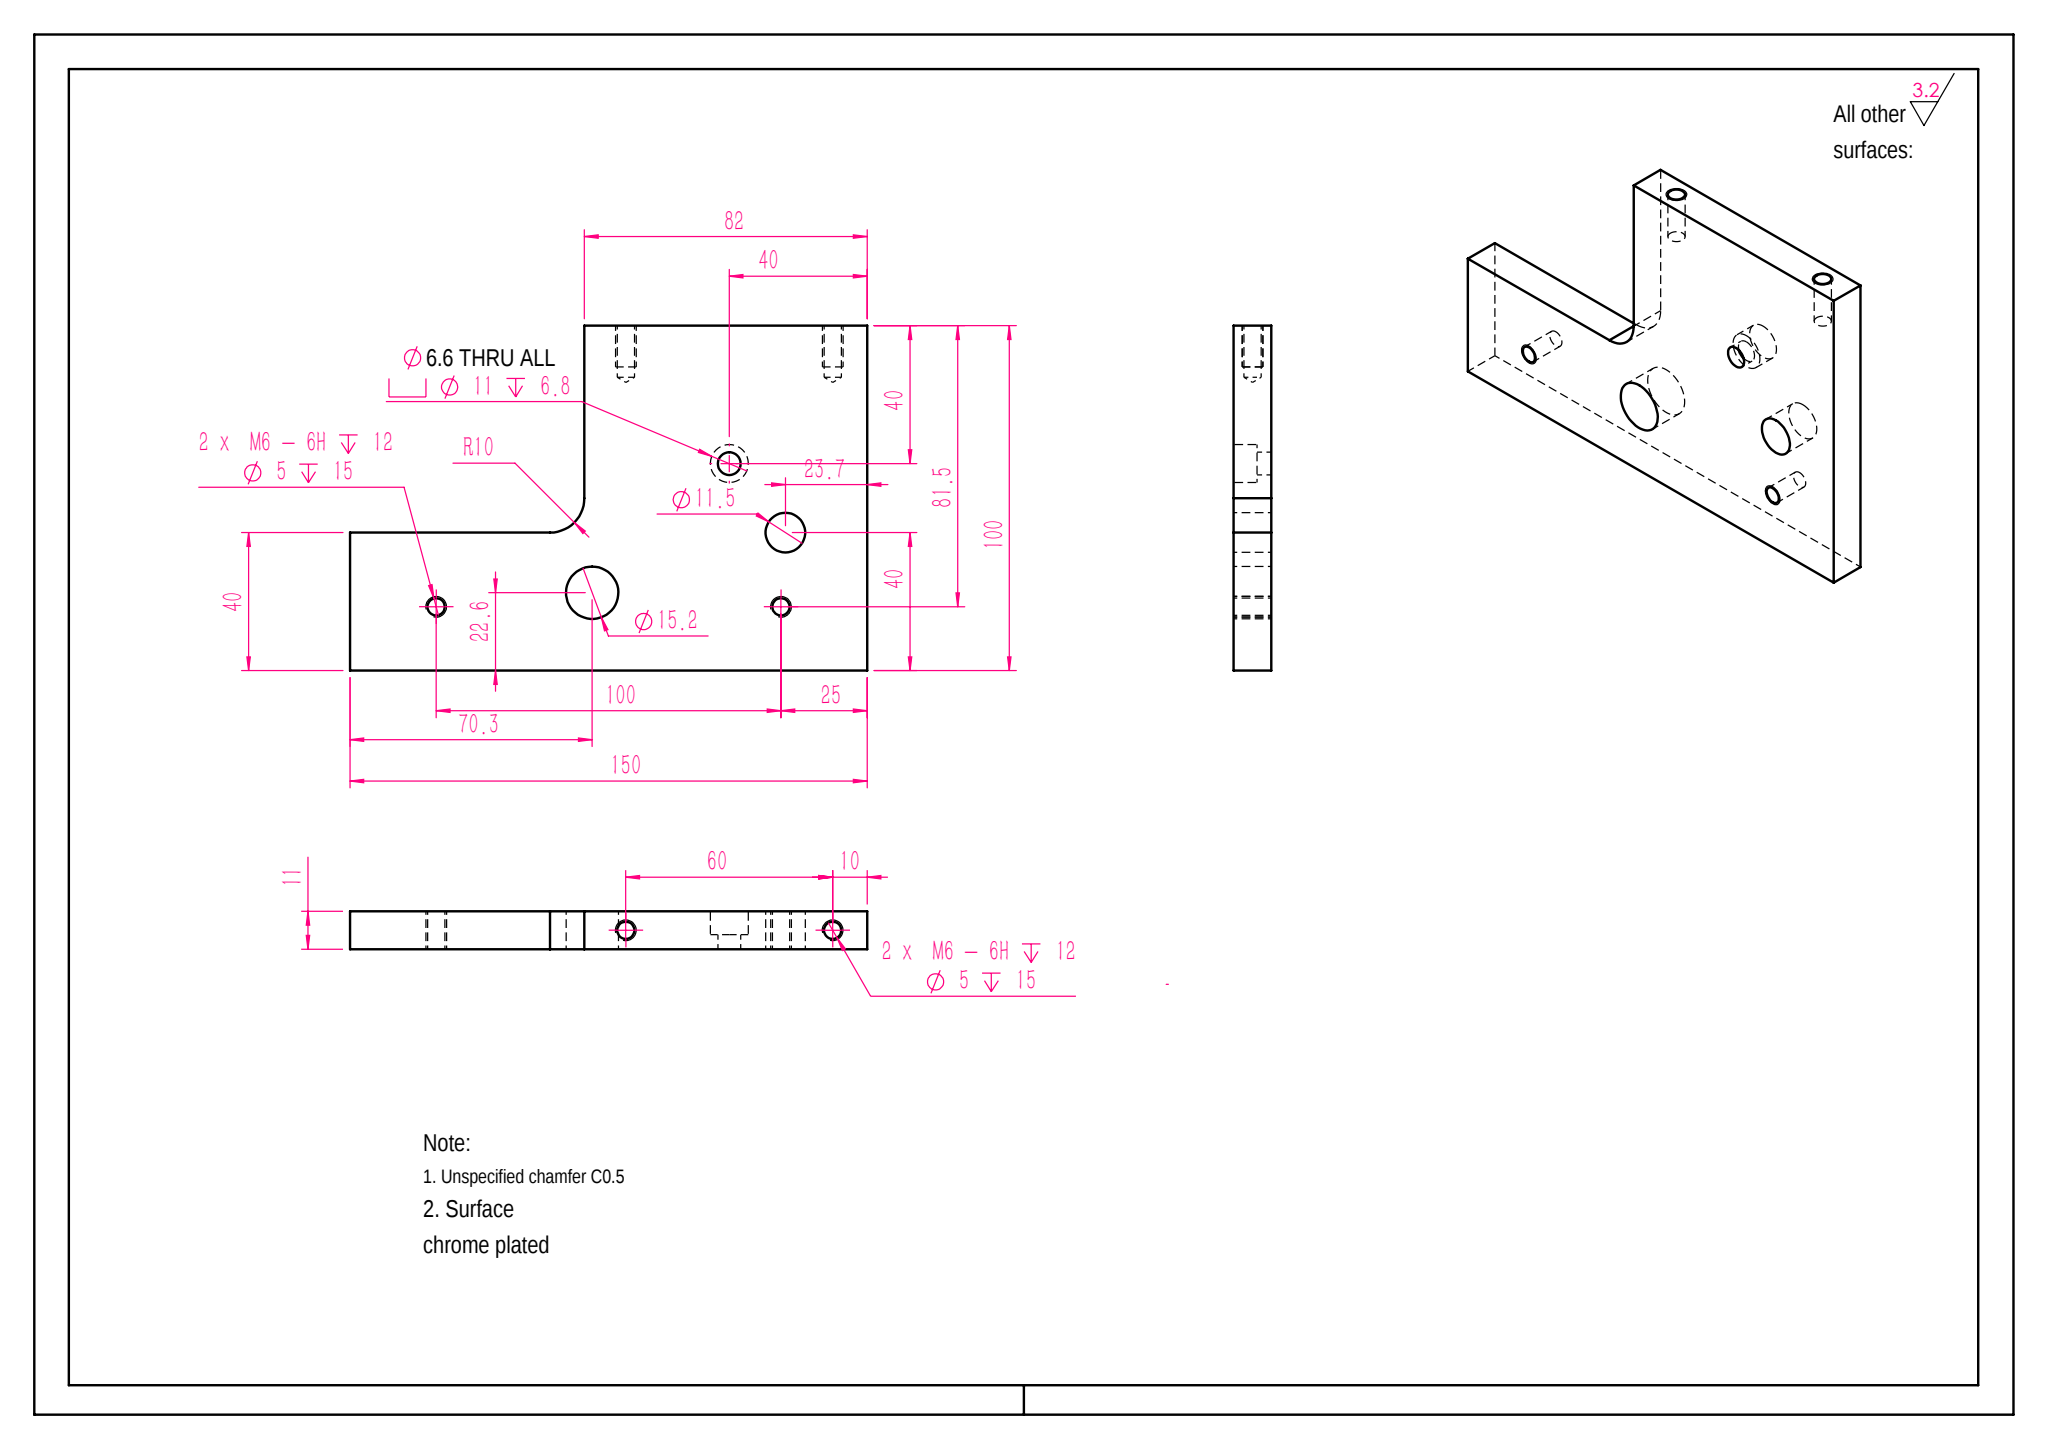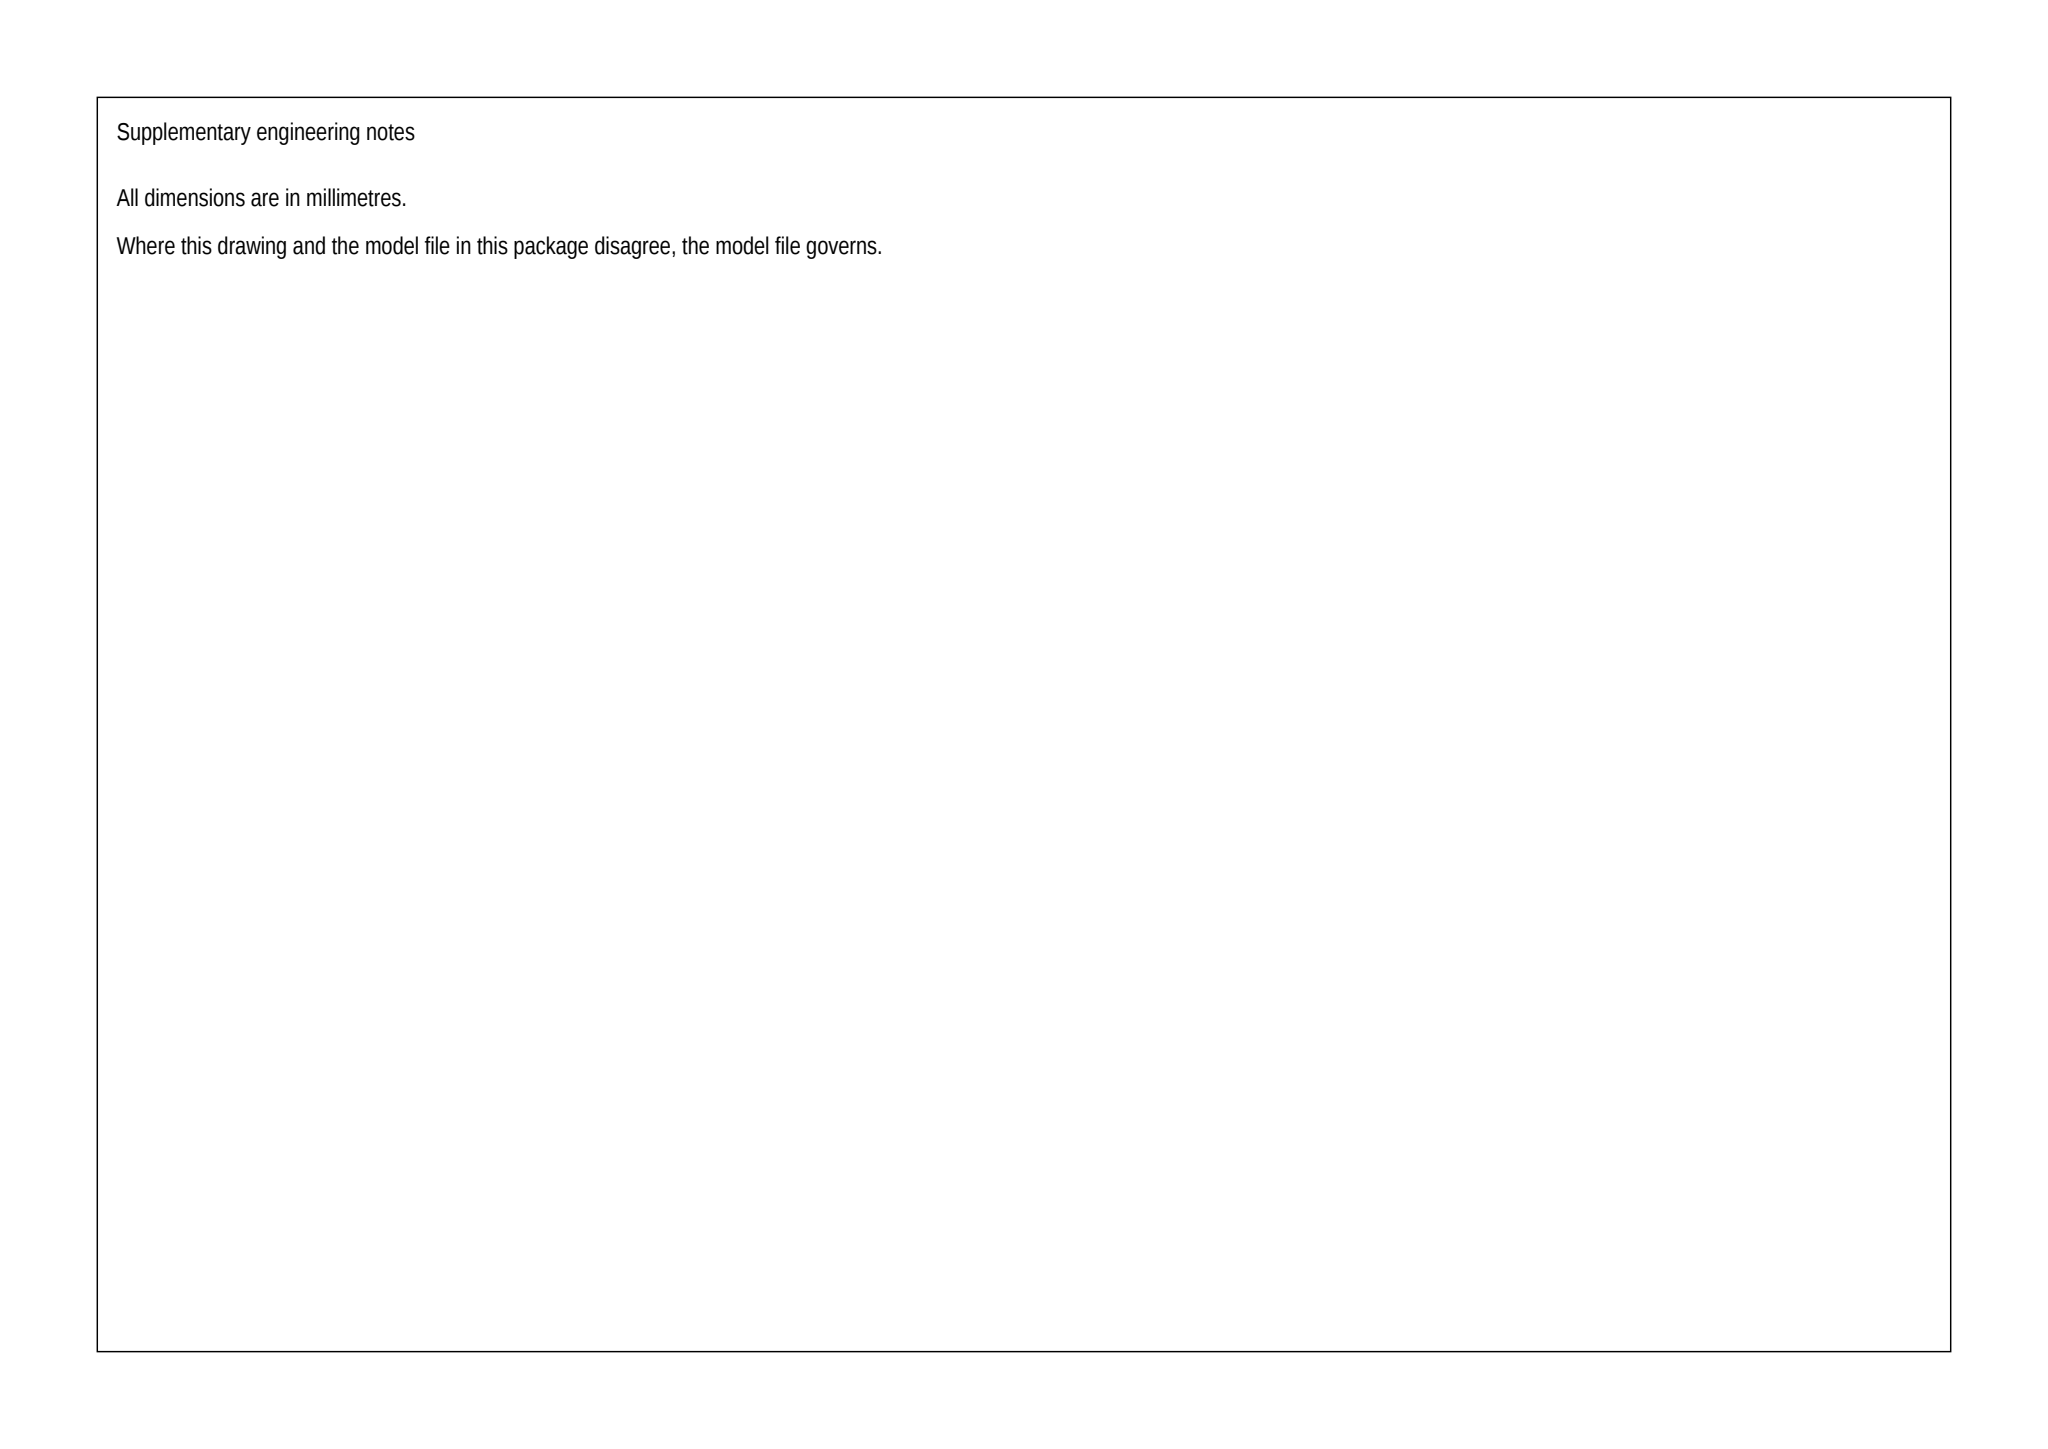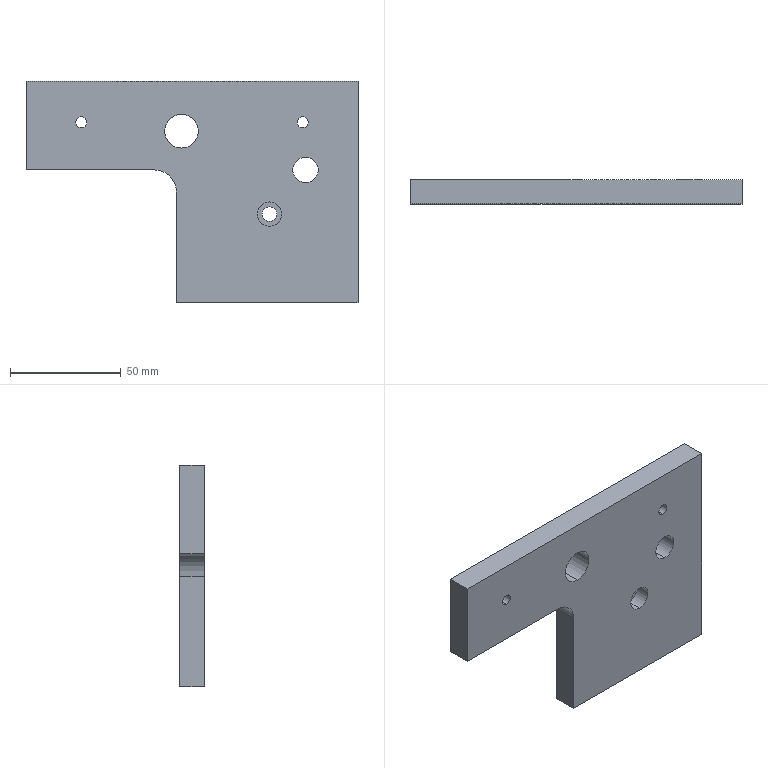Part | SolidWorks | mm | 1 solid | 30 faces | box 150 x 11 x 100 mm | volume 115394 mm3 | cylinder 17 | plane 9 | cone 4 | commonest cylinder face diameters 5 x8 15.175 x2 11.496 x2 11 x2 6.6 x2 20 x1
build123d program:
from build123d import *

# Parameters (mm, degrees)
SKETCH1_W                                            = 150
SKETCH1_H                                            = 100
BOSS_EXTRUDE1_DEPTH                                  = 11
CUT_EXTRUDE1_REACH                                   = 92.807
M6_TAPPED_HOLE1_D                                    = 5
M6_TAPPED_HOLE1_DEPTH                                = 15
M6_TAPPED_HOLE1_TIP                                  = 1.502
M6_TAPPED_HOLE2_D                                    = 5
M6_TAPPED_HOLE2_DEPTH                                = 15
M6_TAPPED_HOLE2_TIP                                  = 1.502
HOLE_SIZE_ACCORDING_TO_HEX_SOCKET_HEAD_C_D           = 6.6
HOLE_SIZE_ACCORDING_TO_HEX_SOCKET_HEAD_C_CBORE_D     = 11
HOLE_SIZE_ACCORDING_TO_HEX_SOCKET_HEAD_C_CBORE_DEPTH = 6.8
SKETCH9_R                                            = 7.588
SKETCH9_R_2                                          = 5.748
CUT_EXTRUDE2_DEPTH                                   = 80


with BuildPart() as part:
    # Sketch1 → Boss-Extrude1 (new body)
    with BuildSketch(Plane(origin=(0, 0, 0), x_dir=(1, 0, 0), z_dir=(0, 1, 0))):
        Rectangle(SKETCH1_W, SKETCH1_H)
    extrude(amount=BOSS_EXTRUDE1_DEPTH)

    # Sketch2 → Cut-Extrude1 (cut, up to next)
    with BuildSketch(Plane(origin=(0, 11, 0), x_dir=(1, 0, 0), z_dir=(0, 1, 0)), mode=Mode.PRIVATE) as cut_extrude1_sk1:
        with BuildLine():
            Line((-7, 50), (-75, 50))
            Line((-75, 50), (-75, -10))
            Line((-75, -10), (-17, -10))
            ThreePointArc((-17, -10), (-9.929, -7.071), (-7, 0))
            Line((-7, 0), (-7, 50))
        make_face()
    cut_extrude1_tool1 = extrude(cut_extrude1_sk1.sketch, amount=-CUT_EXTRUDE1_REACH, mode=Mode.PRIVATE) & part.part
    add(cut_extrude1_tool1.solids().sort_by_distance((-41.168, 11, -20.147))[0], mode=Mode.SUBTRACT)

    # M6 Tapped Hole1
    with Locations(Plane(origin=(0, 0, -50), x_dir=(-1, 0, 0), z_dir=(0, 0, -1))):
        with Locations((-65, 5.5), (-5, 5.5)):
            Hole(M6_TAPPED_HOLE1_D / 2, depth=M6_TAPPED_HOLE1_DEPTH)
            with Locations((0, 0, -(M6_TAPPED_HOLE1_DEPTH + M6_TAPPED_HOLE1_TIP / 2))):  # 118° drill point
                Cone(0, M6_TAPPED_HOLE1_D / 2, M6_TAPPED_HOLE1_TIP, mode=Mode.SUBTRACT)

    # M6 Tapped Hole2
    with Locations(Plane(origin=(0, 11, 0), x_dir=(1, 0, 0), z_dir=(0, 1, 0))):
        with Locations((-50, -31.5), (50, -31.5)):
            Hole(M6_TAPPED_HOLE2_D / 2, depth=M6_TAPPED_HOLE2_DEPTH)
            with Locations((0, 0, -(M6_TAPPED_HOLE2_DEPTH + M6_TAPPED_HOLE2_TIP / 2))):  # 118° drill point
                Cone(0, M6_TAPPED_HOLE2_D / 2, M6_TAPPED_HOLE2_TIP, mode=Mode.SUBTRACT)

    # Hole Size according to Hex Socket Head C (through all)
    with Locations(Plane(origin=(0, 0, 0), x_dir=(-1, 0, 0), z_dir=(0, -1, 0))):
        with Locations((-35, 10)):
            CounterBoreHole(HOLE_SIZE_ACCORDING_TO_HEX_SOCKET_HEAD_C_D / 2, HOLE_SIZE_ACCORDING_TO_HEX_SOCKET_HEAD_C_CBORE_D / 2, HOLE_SIZE_ACCORDING_TO_HEX_SOCKET_HEAD_C_CBORE_DEPTH)

    # Sketch9 → Cut-Extrude2 (cut)
    with BuildSketch(Plane(origin=(0, 0, 0), x_dir=(-1, 0, 0), z_dir=(0, -1, 0))):
        with Locations(Location((4.74, -27.424, 0), (0, 0, 90))):
            Circle(SKETCH9_R)
        with Locations(Location((-51.293, -9.988, 0), (0, 0, 90))):
            Circle(SKETCH9_R_2)
    extrude(amount=-CUT_EXTRUDE2_DEPTH, mode=Mode.SUBTRACT)


solid = part.part